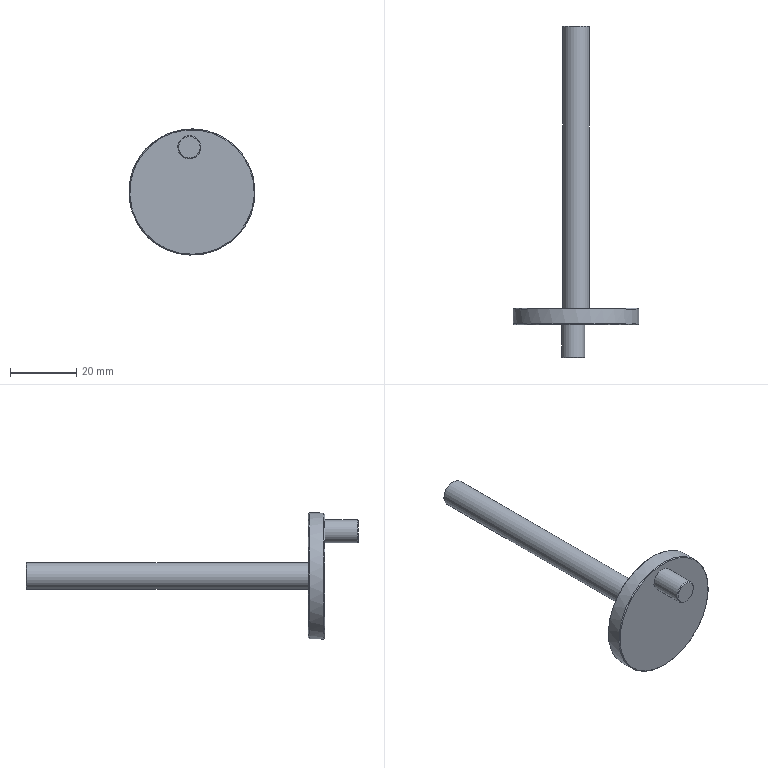Component | NX | CRANKSHAFT | 1 solid | 11 faces | box 38 x 100 x 38 mm | volume 10319 mm3 | plane 4 | cone 4 | cylinder 3 | commonest cylinder face diameters 38 x1 8 x1 7 x1
STEP:
#1=CARTESIAN_POINT('',(0.,0.,0.));
#2=DIRECTION('',(0.,0.,1.));
#3=DIRECTION('',(1.,0.,0.));
#4=AXIS2_PLACEMENT_3D('',#1,#2,#3);
#5=CARTESIAN_POINT('',(18.717,-24.75,42.11));
#6=VERTEX_POINT('',#5);
#7=CARTESIAN_POINT('',(0.,-24.75,41.));
#8=DIRECTION('',(0.,1.,0.));
#9=DIRECTION('',(0.9982,0.,0.05921));
#10=AXIS2_PLACEMENT_3D('',#7,#8,#9);
#11=CIRCLE('',#10,18.75);
#12=CARTESIAN_POINT('',(0.,-24.75,41.));
#13=DIRECTION('',(0.,1.,0.));
#14=DIRECTION('',(0.9982,0.,0.05921));
#15=AXIS2_PLACEMENT_3D('',#12,#13,#14);
#16=PLANE('',#15);
#17=CARTESIAN_POINT('',(0.,0.));
#18=DIRECTION('',(1.,0.));
#19=AXIS2_PLACEMENT_2D('',#17,#18);
#20=CIRCLE('',#19,18.75);
#21=(GEOMETRIC_REPRESENTATION_CONTEXT(2)PARAMETRIC_REPRESENTATION_CONTEXT()REPRESENTATION_CONTEXT('',''));
#22=DEFINITIONAL_REPRESENTATION('',(#20),#21);
#23=PCURVE('',#16,#22);
#24=CARTESIAN_POINT('',(0.,-25.,41.));
#25=DIRECTION('',(0.,-1.,0.));
#26=DIRECTION('',(-0.9982,0.,-0.05921));
#27=AXIS2_PLACEMENT_3D('',#24,#25,#26);
#28=CONICAL_SURFACE('',#27,19.,0.7854);
#29=CARTESIAN_POINT('',(9.425,-0.25));
#30=DIRECTION('',(-1.,0.));
#31=VECTOR('',#30,1.);
#32=LINE('',#29,#31);
#33=(GEOMETRIC_REPRESENTATION_CONTEXT(2)PARAMETRIC_REPRESENTATION_CONTEXT()REPRESENTATION_CONTEXT('',''));
#34=DEFINITIONAL_REPRESENTATION('',(#32),#33);
#35=PCURVE('',#28,#34);
#36=SURFACE_CURVE('',#11,(#23,#35),.PCURVE_S1.);
#37=EDGE_CURVE('',#6,#6,#36,.T.);
#38=ORIENTED_EDGE('',*,*,#37,.T.);
#39=EDGE_LOOP('',(#38));
#40=FACE_BOUND('',#39,.T.);
#41=CARTESIAN_POINT('',(3.993,-24.75,41.237));
#42=VERTEX_POINT('',#41);
#43=CARTESIAN_POINT('',(0.,-24.75,41.));
#44=DIRECTION('',(0.,1.,0.));
#45=DIRECTION('',(0.9982,0.,0.05921));
#46=AXIS2_PLACEMENT_3D('',#43,#44,#45);
#47=CIRCLE('',#46,4.);
#48=CARTESIAN_POINT('',(-0.,-0.));
#49=DIRECTION('',(1.,-0.));
#50=AXIS2_PLACEMENT_2D('',#48,#49);
#51=CIRCLE('',#50,4.);
#52=(GEOMETRIC_REPRESENTATION_CONTEXT(2)PARAMETRIC_REPRESENTATION_CONTEXT()REPRESENTATION_CONTEXT('',''));
#53=DEFINITIONAL_REPRESENTATION('',(#51),#52);
#54=PCURVE('',#16,#53);
#55=CARTESIAN_POINT('',(0.,-24.75,41.));
#56=DIRECTION('',(0.,1.,0.));
#57=DIRECTION('',(0.9982,0.,0.05921));
#58=AXIS2_PLACEMENT_3D('',#55,#56,#57);
#59=CYLINDRICAL_SURFACE('',#58,4.);
#60=CARTESIAN_POINT('',(0.,0.));
#61=DIRECTION('',(1.,0.));
#62=VECTOR('',#61,1.);
#63=LINE('',#60,#62);
#64=(GEOMETRIC_REPRESENTATION_CONTEXT(2)PARAMETRIC_REPRESENTATION_CONTEXT()REPRESENTATION_CONTEXT('',''));
#65=DEFINITIONAL_REPRESENTATION('',(#63),#64);
#66=PCURVE('',#59,#65);
#67=SURFACE_CURVE('',#47,(#54,#66),.PCURVE_S1.);
#68=EDGE_CURVE('',#42,#42,#67,.T.);
#69=ORIENTED_EDGE('',*,*,#68,.F.);
#70=EDGE_LOOP('',(#69));
#71=FACE_BOUND('',#70,.T.);
#72=ADVANCED_FACE('',(#40,#71),#16,.T.);
#73=CARTESIAN_POINT('',(-18.717,-29.75,39.89));
#74=VERTEX_POINT('',#73);
#75=CARTESIAN_POINT('',(0.,-29.75,41.));
#76=DIRECTION('',(0.,-1.,0.));
#77=DIRECTION('',(-0.9982,0.,-0.05921));
#78=AXIS2_PLACEMENT_3D('',#75,#76,#77);
#79=CIRCLE('',#78,18.75);
#80=CARTESIAN_POINT('',(0.,-29.75,41.));
#81=DIRECTION('',(0.,-1.,0.));
#82=DIRECTION('',(-0.9982,0.,-0.05921));
#83=AXIS2_PLACEMENT_3D('',#80,#81,#82);
#84=PLANE('',#83);
#85=CARTESIAN_POINT('',(0.,0.));
#86=DIRECTION('',(1.,0.));
#87=AXIS2_PLACEMENT_2D('',#85,#86);
#88=CIRCLE('',#87,18.75);
#89=(GEOMETRIC_REPRESENTATION_CONTEXT(2)PARAMETRIC_REPRESENTATION_CONTEXT()REPRESENTATION_CONTEXT('',''));
#90=DEFINITIONAL_REPRESENTATION('',(#88),#89);
#91=PCURVE('',#84,#90);
#92=CARTESIAN_POINT('',(0.,-29.5,41.));
#93=DIRECTION('',(0.,1.,0.));
#94=DIRECTION('',(0.9982,0.,0.05921));
#95=AXIS2_PLACEMENT_3D('',#92,#93,#94);
#96=CONICAL_SURFACE('',#95,19.,0.7854);
#97=CARTESIAN_POINT('',(9.425,-0.25));
#98=DIRECTION('',(-1.,0.));
#99=VECTOR('',#98,1.);
#100=LINE('',#97,#99);
#101=(GEOMETRIC_REPRESENTATION_CONTEXT(2)PARAMETRIC_REPRESENTATION_CONTEXT()REPRESENTATION_CONTEXT('',''));
#102=DEFINITIONAL_REPRESENTATION('',(#100),#101);
#103=PCURVE('',#96,#102);
#104=SURFACE_CURVE('',#79,(#91,#103),.PCURVE_S1.);
#105=EDGE_CURVE('',#74,#74,#104,.T.);
#106=ORIENTED_EDGE('',*,*,#105,.T.);
#107=EDGE_LOOP('',(#106));
#108=FACE_BOUND('',#107,.T.);
#109=CARTESIAN_POINT('',(2.694,-29.75,54.684));
#110=VERTEX_POINT('',#109);
#111=CARTESIAN_POINT('',(-0.7994,-29.75,54.476));
#112=DIRECTION('',(0.,1.,0.));
#113=DIRECTION('',(0.9982,0.,0.05921));
#114=AXIS2_PLACEMENT_3D('',#111,#112,#113);
#115=CIRCLE('',#114,3.5);
#116=CARTESIAN_POINT('',(-3.5,-13.5));
#117=CARTESIAN_POINT('',(-3.5,-7.438));
#118=CARTESIAN_POINT('',(1.75,-10.469));
#119=CARTESIAN_POINT('',(7.,-13.5));
#120=CARTESIAN_POINT('',(1.75,-16.531));
#121=CARTESIAN_POINT('',(-3.5,-19.562));
#122=CARTESIAN_POINT('',(-3.5,-13.5));
#123=(BOUNDED_CURVE()B_SPLINE_CURVE(2,(#116,#117,#118,#119,#120,#121,#122),.UNSPECIFIED.,.T.,.F.)B_SPLINE_CURVE_WITH_KNOTS((1,2,2,2,2,1),(-2.094,0.,2.094,4.189,6.283,8.378),.UNSPECIFIED.)CURVE()GEOMETRIC_REPRESENTATION_ITEM()RATIONAL_B_SPLINE_CURVE((1.,0.5,1.,0.5,1.,0.5,1.))REPRESENTATION_ITEM(''));
#124=(GEOMETRIC_REPRESENTATION_CONTEXT(2)PARAMETRIC_REPRESENTATION_CONTEXT()REPRESENTATION_CONTEXT('',''));
#125=DEFINITIONAL_REPRESENTATION('',(#123),#124);
#126=PCURVE('',#84,#125);
#127=CARTESIAN_POINT('',(-0.7994,-39.75,54.476));
#128=DIRECTION('',(0.,1.,0.));
#129=DIRECTION('',(0.9982,0.,0.05921));
#130=AXIS2_PLACEMENT_3D('',#127,#128,#129);
#131=CYLINDRICAL_SURFACE('',#130,3.5);
#132=CARTESIAN_POINT('',(0.,10.));
#133=DIRECTION('',(1.,0.));
#134=VECTOR('',#133,1.);
#135=LINE('',#132,#134);
#136=(GEOMETRIC_REPRESENTATION_CONTEXT(2)PARAMETRIC_REPRESENTATION_CONTEXT()REPRESENTATION_CONTEXT('',''));
#137=DEFINITIONAL_REPRESENTATION('',(#135),#136);
#138=PCURVE('',#131,#137);
#139=SURFACE_CURVE('',#115,(#126,#138),.PCURVE_S1.);
#140=EDGE_CURVE('',#110,#110,#139,.T.);
#141=ORIENTED_EDGE('',*,*,#140,.T.);
#142=EDGE_LOOP('',(#141));
#143=FACE_BOUND('',#142,.T.);
#144=ADVANCED_FACE('',(#108,#143),#84,.T.);
#145=CARTESIAN_POINT('',(18.967,-25.,42.125));
#146=VERTEX_POINT('',#145);
#147=CARTESIAN_POINT('',(0.,-25.,41.));
#148=DIRECTION('',(0.,-1.,0.));
#149=DIRECTION('',(0.9982,0.,0.05921));
#150=AXIS2_PLACEMENT_3D('',#147,#148,#149);
#151=CIRCLE('',#150,19.);
#152=CARTESIAN_POINT('',(0.,-29.75,41.));
#153=DIRECTION('',(0.,1.,0.));
#154=DIRECTION('',(0.9982,0.,0.05921));
#155=AXIS2_PLACEMENT_3D('',#152,#153,#154);
#156=CYLINDRICAL_SURFACE('',#155,19.);
#157=CARTESIAN_POINT('',(6.283,4.75));
#158=DIRECTION('',(-1.,0.));
#159=VECTOR('',#158,1.);
#160=LINE('',#157,#159);
#161=(GEOMETRIC_REPRESENTATION_CONTEXT(2)PARAMETRIC_REPRESENTATION_CONTEXT()REPRESENTATION_CONTEXT('',''));
#162=DEFINITIONAL_REPRESENTATION('',(#160),#161);
#163=PCURVE('',#156,#162);
#164=CARTESIAN_POINT('',(3.142,0.));
#165=DIRECTION('',(1.,0.));
#166=VECTOR('',#165,1.);
#167=LINE('',#164,#166);
#168=(GEOMETRIC_REPRESENTATION_CONTEXT(2)PARAMETRIC_REPRESENTATION_CONTEXT()REPRESENTATION_CONTEXT('',''));
#169=DEFINITIONAL_REPRESENTATION('',(#167),#168);
#170=PCURVE('',#28,#169);
#171=SURFACE_CURVE('',#151,(#163,#170),.PCURVE_S1.);
#172=EDGE_CURVE('',#146,#146,#171,.T.);
#173=ORIENTED_EDGE('',*,*,#172,.T.);
#174=CARTESIAN_POINT('',(18.967,-29.5,42.125));
#175=VERTEX_POINT('',#174);
#176=CARTESIAN_POINT('',(18.967,-29.5,42.125));
#177=CARTESIAN_POINT('',(18.967,-25.,42.125));
#178=B_SPLINE_CURVE_WITH_KNOTS('',1,(#176,#177),.UNSPECIFIED.,.F.,.F.,(2,2),(0.25,4.75),.PIECEWISE_BEZIER_KNOTS.);
#179=CARTESIAN_POINT('',(0.,0.));
#180=DIRECTION('',(0.,1.));
#181=VECTOR('',#180,1.);
#182=LINE('',#179,#181);
#183=(GEOMETRIC_REPRESENTATION_CONTEXT(2)PARAMETRIC_REPRESENTATION_CONTEXT()REPRESENTATION_CONTEXT('',''));
#184=DEFINITIONAL_REPRESENTATION('',(#182),#183);
#185=PCURVE('',#156,#184);
#186=CARTESIAN_POINT('',(6.283,0.));
#187=DIRECTION('',(0.,1.));
#188=VECTOR('',#187,1.);
#189=LINE('',#186,#188);
#190=(GEOMETRIC_REPRESENTATION_CONTEXT(2)PARAMETRIC_REPRESENTATION_CONTEXT()REPRESENTATION_CONTEXT('',''));
#191=DEFINITIONAL_REPRESENTATION('',(#189),#190);
#192=PCURVE('',#156,#191);
#193=SEAM_CURVE('',#178,(#185,#192),.PCURVE_S1.);
#194=EDGE_CURVE('',#175,#146,#193,.T.);
#195=ORIENTED_EDGE('',*,*,#194,.F.);
#196=CARTESIAN_POINT('',(-18.967,-29.5,39.875));
#197=VERTEX_POINT('',#196);
#198=CARTESIAN_POINT('',(0.,-29.5,41.));
#199=DIRECTION('',(0.,1.,0.));
#200=DIRECTION('',(-0.9982,0.,-0.05921));
#201=AXIS2_PLACEMENT_3D('',#198,#199,#200);
#202=CIRCLE('',#201,19.);
#203=CARTESIAN_POINT('',(-3.142,0.25));
#204=DIRECTION('',(1.,0.));
#205=VECTOR('',#204,1.);
#206=LINE('',#203,#205);
#207=(GEOMETRIC_REPRESENTATION_CONTEXT(2)PARAMETRIC_REPRESENTATION_CONTEXT()REPRESENTATION_CONTEXT('',''));
#208=DEFINITIONAL_REPRESENTATION('',(#206),#207);
#209=PCURVE('',#156,#208);
#210=CARTESIAN_POINT('',(3.142,0.));
#211=DIRECTION('',(1.,0.));
#212=VECTOR('',#211,1.);
#213=LINE('',#210,#212);
#214=(GEOMETRIC_REPRESENTATION_CONTEXT(2)PARAMETRIC_REPRESENTATION_CONTEXT()REPRESENTATION_CONTEXT('',''));
#215=DEFINITIONAL_REPRESENTATION('',(#213),#214);
#216=PCURVE('',#96,#215);
#217=SURFACE_CURVE('',#202,(#209,#216),.PCURVE_S1.);
#218=EDGE_CURVE('',#175,#197,#217,.T.);
#219=ORIENTED_EDGE('',*,*,#218,.T.);
#220=CARTESIAN_POINT('',(0.,-29.5,41.));
#221=DIRECTION('',(0.,1.,0.));
#222=DIRECTION('',(-0.9982,0.,-0.05921));
#223=AXIS2_PLACEMENT_3D('',#220,#221,#222);
#224=CIRCLE('',#223,19.);
#225=CARTESIAN_POINT('',(3.142,0.25));
#226=DIRECTION('',(1.,0.));
#227=VECTOR('',#226,1.);
#228=LINE('',#225,#227);
#229=(GEOMETRIC_REPRESENTATION_CONTEXT(2)PARAMETRIC_REPRESENTATION_CONTEXT()REPRESENTATION_CONTEXT('',''));
#230=DEFINITIONAL_REPRESENTATION('',(#228),#229);
#231=PCURVE('',#156,#230);
#232=CARTESIAN_POINT('',(3.142,0.));
#233=DIRECTION('',(1.,-0.));
#234=VECTOR('',#233,1.);
#235=LINE('',#232,#234);
#236=(GEOMETRIC_REPRESENTATION_CONTEXT(2)PARAMETRIC_REPRESENTATION_CONTEXT()REPRESENTATION_CONTEXT('',''));
#237=DEFINITIONAL_REPRESENTATION('',(#235),#236);
#238=PCURVE('',#96,#237);
#239=SURFACE_CURVE('',#224,(#231,#238),.PCURVE_S1.);
#240=EDGE_CURVE('',#197,#175,#239,.T.);
#241=ORIENTED_EDGE('',*,*,#240,.T.);
#242=ORIENTED_EDGE('',*,*,#194,.T.);
#243=EDGE_LOOP('',(#173,#195,#219,#241,#242));
#244=FACE_BOUND('',#243,.T.);
#245=ADVANCED_FACE('',(#244),#156,.T.);
#246=CARTESIAN_POINT('',(3.743,60.25,41.222));
#247=VERTEX_POINT('',#246);
#248=CARTESIAN_POINT('',(0.,60.25,41.));
#249=DIRECTION('',(0.,1.,0.));
#250=DIRECTION('',(0.9982,0.,0.05921));
#251=AXIS2_PLACEMENT_3D('',#248,#249,#250);
#252=CIRCLE('',#251,3.75);
#253=CARTESIAN_POINT('',(0.,60.25,41.));
#254=DIRECTION('',(0.,1.,0.));
#255=DIRECTION('',(0.9982,0.,0.05921));
#256=AXIS2_PLACEMENT_3D('',#253,#254,#255);
#257=PLANE('',#256);
#258=CARTESIAN_POINT('',(0.,0.));
#259=DIRECTION('',(1.,-0.));
#260=AXIS2_PLACEMENT_2D('',#258,#259);
#261=CIRCLE('',#260,3.75);
#262=(GEOMETRIC_REPRESENTATION_CONTEXT(2)PARAMETRIC_REPRESENTATION_CONTEXT()REPRESENTATION_CONTEXT('',''));
#263=DEFINITIONAL_REPRESENTATION('',(#261),#262);
#264=PCURVE('',#257,#263);
#265=CARTESIAN_POINT('',(0.,60.25,41.));
#266=DIRECTION('',(0.,-1.,0.));
#267=DIRECTION('',(-0.9982,0.,-0.05921));
#268=AXIS2_PLACEMENT_3D('',#265,#266,#267);
#269=CONICAL_SURFACE('',#268,3.75,0.7854);
#270=CARTESIAN_POINT('',(9.425,0.));
#271=DIRECTION('',(-1.,0.));
#272=VECTOR('',#271,1.);
#273=LINE('',#270,#272);
#274=(GEOMETRIC_REPRESENTATION_CONTEXT(2)PARAMETRIC_REPRESENTATION_CONTEXT()REPRESENTATION_CONTEXT('',''));
#275=DEFINITIONAL_REPRESENTATION('',(#273),#274);
#276=PCURVE('',#269,#275);
#277=SURFACE_CURVE('',#252,(#264,#276),.PCURVE_S1.);
#278=EDGE_CURVE('',#247,#247,#277,.T.);
#279=ORIENTED_EDGE('',*,*,#278,.T.);
#280=EDGE_LOOP('',(#279));
#281=FACE_BOUND('',#280,.T.);
#282=ADVANCED_FACE('',(#281),#257,.T.);
#283=CARTESIAN_POINT('',(3.993,60.,41.237));
#284=VERTEX_POINT('',#283);
#285=CARTESIAN_POINT('',(0.,60.,41.));
#286=DIRECTION('',(0.,-1.,0.));
#287=DIRECTION('',(0.9982,0.,0.05921));
#288=AXIS2_PLACEMENT_3D('',#285,#286,#287);
#289=CIRCLE('',#288,4.);
#290=CARTESIAN_POINT('',(6.283,84.75));
#291=DIRECTION('',(-1.,0.));
#292=VECTOR('',#291,1.);
#293=LINE('',#290,#292);
#294=(GEOMETRIC_REPRESENTATION_CONTEXT(2)PARAMETRIC_REPRESENTATION_CONTEXT()REPRESENTATION_CONTEXT('',''));
#295=DEFINITIONAL_REPRESENTATION('',(#293),#294);
#296=PCURVE('',#59,#295);
#297=CARTESIAN_POINT('',(3.142,0.25));
#298=DIRECTION('',(1.,0.));
#299=VECTOR('',#298,1.);
#300=LINE('',#297,#299);
#301=(GEOMETRIC_REPRESENTATION_CONTEXT(2)PARAMETRIC_REPRESENTATION_CONTEXT()REPRESENTATION_CONTEXT('',''));
#302=DEFINITIONAL_REPRESENTATION('',(#300),#301);
#303=PCURVE('',#269,#302);
#304=SURFACE_CURVE('',#289,(#296,#303),.PCURVE_S1.);
#305=EDGE_CURVE('',#284,#284,#304,.T.);
#306=ORIENTED_EDGE('',*,*,#305,.T.);
#307=CARTESIAN_POINT('',(3.993,-24.75,41.237));
#308=CARTESIAN_POINT('',(3.993,60.,41.237));
#309=B_SPLINE_CURVE_WITH_KNOTS('',1,(#307,#308),.UNSPECIFIED.,.F.,.F.,(2,2),(0.,84.75),.PIECEWISE_BEZIER_KNOTS.);
#310=CARTESIAN_POINT('',(0.,0.));
#311=DIRECTION('',(0.,1.));
#312=VECTOR('',#311,1.);
#313=LINE('',#310,#312);
#314=(GEOMETRIC_REPRESENTATION_CONTEXT(2)PARAMETRIC_REPRESENTATION_CONTEXT()REPRESENTATION_CONTEXT('',''));
#315=DEFINITIONAL_REPRESENTATION('',(#313),#314);
#316=PCURVE('',#59,#315);
#317=CARTESIAN_POINT('',(6.283,0.));
#318=DIRECTION('',(0.,1.));
#319=VECTOR('',#318,1.);
#320=LINE('',#317,#319);
#321=(GEOMETRIC_REPRESENTATION_CONTEXT(2)PARAMETRIC_REPRESENTATION_CONTEXT()REPRESENTATION_CONTEXT('',''));
#322=DEFINITIONAL_REPRESENTATION('',(#320),#321);
#323=PCURVE('',#59,#322);
#324=SEAM_CURVE('',#309,(#316,#323),.PCURVE_S1.);
#325=EDGE_CURVE('',#42,#284,#324,.T.);
#326=ORIENTED_EDGE('',*,*,#325,.F.);
#327=ORIENTED_EDGE('',*,*,#68,.T.);
#328=ORIENTED_EDGE('',*,*,#325,.T.);
#329=EDGE_LOOP('',(#306,#326,#327,#328));
#330=FACE_BOUND('',#329,.T.);
#331=ADVANCED_FACE('',(#330),#59,.T.);
#332=CARTESIAN_POINT('',(2.694,-39.5,54.684));
#333=VERTEX_POINT('',#332);
#334=CARTESIAN_POINT('',(-0.7994,-39.5,54.476));
#335=DIRECTION('',(0.,1.,0.));
#336=DIRECTION('',(0.9982,0.,0.05921));
#337=AXIS2_PLACEMENT_3D('',#334,#335,#336);
#338=CIRCLE('',#337,3.5);
#339=CARTESIAN_POINT('',(0.,0.25));
#340=DIRECTION('',(1.,0.));
#341=VECTOR('',#340,1.);
#342=LINE('',#339,#341);
#343=(GEOMETRIC_REPRESENTATION_CONTEXT(2)PARAMETRIC_REPRESENTATION_CONTEXT()REPRESENTATION_CONTEXT('',''));
#344=DEFINITIONAL_REPRESENTATION('',(#342),#343);
#345=PCURVE('',#131,#344);
#346=CARTESIAN_POINT('',(-0.7994,-39.5,54.476));
#347=DIRECTION('',(0.,1.,0.));
#348=DIRECTION('',(0.9982,0.,0.05921));
#349=AXIS2_PLACEMENT_3D('',#346,#347,#348);
#350=CONICAL_SURFACE('',#349,3.5,0.7854);
#351=CARTESIAN_POINT('',(0.,0.));
#352=DIRECTION('',(1.,0.));
#353=VECTOR('',#352,1.);
#354=LINE('',#351,#353);
#355=(GEOMETRIC_REPRESENTATION_CONTEXT(2)PARAMETRIC_REPRESENTATION_CONTEXT()REPRESENTATION_CONTEXT('',''));
#356=DEFINITIONAL_REPRESENTATION('',(#354),#355);
#357=PCURVE('',#350,#356);
#358=SURFACE_CURVE('',#338,(#345,#357),.PCURVE_S1.);
#359=EDGE_CURVE('',#333,#333,#358,.T.);
#360=ORIENTED_EDGE('',*,*,#359,.T.);
#361=CARTESIAN_POINT('',(2.694,-39.5,54.684));
#362=CARTESIAN_POINT('',(2.694,-29.75,54.684));
#363=B_SPLINE_CURVE_WITH_KNOTS('',1,(#361,#362),.UNSPECIFIED.,.F.,.F.,(2,2),(0.25,10.),.PIECEWISE_BEZIER_KNOTS.);
#364=CARTESIAN_POINT('',(6.283,0.));
#365=DIRECTION('',(0.,1.));
#366=VECTOR('',#365,1.);
#367=LINE('',#364,#366);
#368=(GEOMETRIC_REPRESENTATION_CONTEXT(2)PARAMETRIC_REPRESENTATION_CONTEXT()REPRESENTATION_CONTEXT('',''));
#369=DEFINITIONAL_REPRESENTATION('',(#367),#368);
#370=PCURVE('',#131,#369);
#371=CARTESIAN_POINT('',(0.,0.));
#372=DIRECTION('',(0.,1.));
#373=VECTOR('',#372,1.);
#374=LINE('',#371,#373);
#375=(GEOMETRIC_REPRESENTATION_CONTEXT(2)PARAMETRIC_REPRESENTATION_CONTEXT()REPRESENTATION_CONTEXT('',''));
#376=DEFINITIONAL_REPRESENTATION('',(#374),#375);
#377=PCURVE('',#131,#376);
#378=SEAM_CURVE('',#363,(#370,#377),.PCURVE_S1.);
#379=EDGE_CURVE('',#333,#110,#378,.T.);
#380=ORIENTED_EDGE('',*,*,#379,.T.);
#381=ORIENTED_EDGE('',*,*,#140,.F.);
#382=ORIENTED_EDGE('',*,*,#379,.F.);
#383=EDGE_LOOP('',(#360,#380,#381,#382));
#384=FACE_BOUND('',#383,.T.);
#385=ADVANCED_FACE('',(#384),#131,.T.);
#386=CARTESIAN_POINT('',(2.445,-39.75,54.669));
#387=VERTEX_POINT('',#386);
#388=CARTESIAN_POINT('',(-0.7994,-39.75,54.476));
#389=DIRECTION('',(0.,-1.,0.));
#390=DIRECTION('',(0.9982,0.,0.05921));
#391=AXIS2_PLACEMENT_3D('',#388,#389,#390);
#392=CIRCLE('',#391,3.25);
#393=CARTESIAN_POINT('',(-0.7994,-39.75,54.476));
#394=DIRECTION('',(0.,1.,0.));
#395=DIRECTION('',(0.9982,0.,0.05921));
#396=AXIS2_PLACEMENT_3D('',#393,#394,#395);
#397=PLANE('',#396);
#398=CARTESIAN_POINT('',(3.25,-0.));
#399=CARTESIAN_POINT('',(3.25,-5.629));
#400=CARTESIAN_POINT('',(-1.625,-2.815));
#401=CARTESIAN_POINT('',(-6.5,0.));
#402=CARTESIAN_POINT('',(-1.625,2.815));
#403=CARTESIAN_POINT('',(3.25,5.629));
#404=CARTESIAN_POINT('',(3.25,-0.));
#405=(BOUNDED_CURVE()B_SPLINE_CURVE(2,(#398,#399,#400,#401,#402,#403,#404),.UNSPECIFIED.,.T.,.F.)B_SPLINE_CURVE_WITH_KNOTS((1,2,2,2,2,1),(-2.094,0.,2.094,4.189,6.283,8.378),.UNSPECIFIED.)CURVE()GEOMETRIC_REPRESENTATION_ITEM()RATIONAL_B_SPLINE_CURVE((1.,0.5,1.,0.5,1.,0.5,1.))REPRESENTATION_ITEM(''));
#406=(GEOMETRIC_REPRESENTATION_CONTEXT(2)PARAMETRIC_REPRESENTATION_CONTEXT()REPRESENTATION_CONTEXT('',''));
#407=DEFINITIONAL_REPRESENTATION('',(#405),#406);
#408=PCURVE('',#397,#407);
#409=CARTESIAN_POINT('',(6.283,-0.25));
#410=DIRECTION('',(-1.,0.));
#411=VECTOR('',#410,1.);
#412=LINE('',#409,#411);
#413=(GEOMETRIC_REPRESENTATION_CONTEXT(2)PARAMETRIC_REPRESENTATION_CONTEXT()REPRESENTATION_CONTEXT('',''));
#414=DEFINITIONAL_REPRESENTATION('',(#412),#413);
#415=PCURVE('',#350,#414);
#416=SURFACE_CURVE('',#392,(#408,#415),.PCURVE_S1.);
#417=EDGE_CURVE('',#387,#387,#416,.T.);
#418=ORIENTED_EDGE('',*,*,#417,.T.);
#419=EDGE_LOOP('',(#418));
#420=FACE_BOUND('',#419,.T.);
#421=ADVANCED_FACE('',(#420),#397,.F.);
#422=ORIENTED_EDGE('',*,*,#37,.F.);
#423=CARTESIAN_POINT('',(18.717,-24.75,42.11));
#424=CARTESIAN_POINT('',(18.967,-25.,42.125));
#425=B_SPLINE_CURVE_WITH_KNOTS('',1,(#423,#424),.UNSPECIFIED.,.F.,.F.,(2,2),(-0.3536,0.),.PIECEWISE_BEZIER_KNOTS.);
#426=CARTESIAN_POINT('',(9.425,0.));
#427=DIRECTION('',(0.,1.));
#428=VECTOR('',#427,1.);
#429=LINE('',#426,#428);
#430=(GEOMETRIC_REPRESENTATION_CONTEXT(2)PARAMETRIC_REPRESENTATION_CONTEXT()REPRESENTATION_CONTEXT('',''));
#431=DEFINITIONAL_REPRESENTATION('',(#429),#430);
#432=PCURVE('',#28,#431);
#433=CARTESIAN_POINT('',(3.142,0.));
#434=DIRECTION('',(0.,1.));
#435=VECTOR('',#434,1.);
#436=LINE('',#433,#435);
#437=(GEOMETRIC_REPRESENTATION_CONTEXT(2)PARAMETRIC_REPRESENTATION_CONTEXT()REPRESENTATION_CONTEXT('',''));
#438=DEFINITIONAL_REPRESENTATION('',(#436),#437);
#439=PCURVE('',#28,#438);
#440=SEAM_CURVE('',#425,(#432,#439),.PCURVE_S1.);
#441=EDGE_CURVE('',#6,#146,#440,.T.);
#442=ORIENTED_EDGE('',*,*,#441,.T.);
#443=ORIENTED_EDGE('',*,*,#172,.F.);
#444=ORIENTED_EDGE('',*,*,#441,.F.);
#445=EDGE_LOOP('',(#422,#442,#443,#444));
#446=FACE_BOUND('',#445,.T.);
#447=ADVANCED_FACE('',(#446),#28,.T.);
#448=ORIENTED_EDGE('',*,*,#105,.F.);
#449=CARTESIAN_POINT('',(-18.717,-29.75,39.89));
#450=CARTESIAN_POINT('',(-18.967,-29.5,39.875));
#451=B_SPLINE_CURVE_WITH_KNOTS('',1,(#449,#450),.UNSPECIFIED.,.F.,.F.,(2,2),(-0.3536,0.),.PIECEWISE_BEZIER_KNOTS.);
#452=CARTESIAN_POINT('',(9.425,0.));
#453=DIRECTION('',(0.,1.));
#454=VECTOR('',#453,1.);
#455=LINE('',#452,#454);
#456=(GEOMETRIC_REPRESENTATION_CONTEXT(2)PARAMETRIC_REPRESENTATION_CONTEXT()REPRESENTATION_CONTEXT('',''));
#457=DEFINITIONAL_REPRESENTATION('',(#455),#456);
#458=PCURVE('',#96,#457);
#459=CARTESIAN_POINT('',(3.142,0.));
#460=DIRECTION('',(0.,1.));
#461=VECTOR('',#460,1.);
#462=LINE('',#459,#461);
#463=(GEOMETRIC_REPRESENTATION_CONTEXT(2)PARAMETRIC_REPRESENTATION_CONTEXT()REPRESENTATION_CONTEXT('',''));
#464=DEFINITIONAL_REPRESENTATION('',(#462),#463);
#465=PCURVE('',#96,#464);
#466=SEAM_CURVE('',#451,(#458,#465),.PCURVE_S1.);
#467=EDGE_CURVE('',#74,#197,#466,.T.);
#468=ORIENTED_EDGE('',*,*,#467,.T.);
#469=ORIENTED_EDGE('',*,*,#218,.F.);
#470=ORIENTED_EDGE('',*,*,#240,.F.);
#471=ORIENTED_EDGE('',*,*,#467,.F.);
#472=EDGE_LOOP('',(#448,#468,#469,#470,#471));
#473=FACE_BOUND('',#472,.T.);
#474=ADVANCED_FACE('',(#473),#96,.T.);
#475=ORIENTED_EDGE('',*,*,#305,.F.);
#476=CARTESIAN_POINT('',(3.743,60.25,41.222));
#477=CARTESIAN_POINT('',(3.993,60.,41.237));
#478=B_SPLINE_CURVE_WITH_KNOTS('',1,(#476,#477),.UNSPECIFIED.,.F.,.F.,(2,2),(0.,0.3536),.PIECEWISE_BEZIER_KNOTS.);
#479=CARTESIAN_POINT('',(3.142,0.));
#480=DIRECTION('',(0.,1.));
#481=VECTOR('',#480,1.);
#482=LINE('',#479,#481);
#483=(GEOMETRIC_REPRESENTATION_CONTEXT(2)PARAMETRIC_REPRESENTATION_CONTEXT()REPRESENTATION_CONTEXT('',''));
#484=DEFINITIONAL_REPRESENTATION('',(#482),#483);
#485=PCURVE('',#269,#484);
#486=CARTESIAN_POINT('',(9.425,0.));
#487=DIRECTION('',(0.,1.));
#488=VECTOR('',#487,1.);
#489=LINE('',#486,#488);
#490=(GEOMETRIC_REPRESENTATION_CONTEXT(2)PARAMETRIC_REPRESENTATION_CONTEXT()REPRESENTATION_CONTEXT('',''));
#491=DEFINITIONAL_REPRESENTATION('',(#489),#490);
#492=PCURVE('',#269,#491);
#493=SEAM_CURVE('',#478,(#485,#492),.PCURVE_S1.);
#494=EDGE_CURVE('',#247,#284,#493,.T.);
#495=ORIENTED_EDGE('',*,*,#494,.F.);
#496=ORIENTED_EDGE('',*,*,#278,.F.);
#497=ORIENTED_EDGE('',*,*,#494,.T.);
#498=EDGE_LOOP('',(#475,#495,#496,#497));
#499=FACE_BOUND('',#498,.T.);
#500=ADVANCED_FACE('',(#499),#269,.T.);
#501=ORIENTED_EDGE('',*,*,#417,.F.);
#502=CARTESIAN_POINT('',(2.445,-39.75,54.669));
#503=CARTESIAN_POINT('',(2.694,-39.5,54.684));
#504=B_SPLINE_CURVE_WITH_KNOTS('',1,(#502,#503),.UNSPECIFIED.,.F.,.F.,(2,2),(-0.3536,0.),.PIECEWISE_BEZIER_KNOTS.);
#505=CARTESIAN_POINT('',(6.283,0.));
#506=DIRECTION('',(0.,1.));
#507=VECTOR('',#506,1.);
#508=LINE('',#505,#507);
#509=(GEOMETRIC_REPRESENTATION_CONTEXT(2)PARAMETRIC_REPRESENTATION_CONTEXT()REPRESENTATION_CONTEXT('',''));
#510=DEFINITIONAL_REPRESENTATION('',(#508),#509);
#511=PCURVE('',#350,#510);
#512=CARTESIAN_POINT('',(0.,0.));
#513=DIRECTION('',(0.,1.));
#514=VECTOR('',#513,1.);
#515=LINE('',#512,#514);
#516=(GEOMETRIC_REPRESENTATION_CONTEXT(2)PARAMETRIC_REPRESENTATION_CONTEXT()REPRESENTATION_CONTEXT('',''));
#517=DEFINITIONAL_REPRESENTATION('',(#515),#516);
#518=PCURVE('',#350,#517);
#519=SEAM_CURVE('',#504,(#511,#518),.PCURVE_S1.);
#520=EDGE_CURVE('',#387,#333,#519,.T.);
#521=ORIENTED_EDGE('',*,*,#520,.T.);
#522=ORIENTED_EDGE('',*,*,#359,.F.);
#523=ORIENTED_EDGE('',*,*,#520,.F.);
#524=EDGE_LOOP('',(#501,#521,#522,#523));
#525=FACE_BOUND('',#524,.T.);
#526=ADVANCED_FACE('',(#525),#350,.T.);
#527=CLOSED_SHELL('',(#72,#144,#245,#282,#331,#385,#421,#447,#474,#500,#526));
#528=MANIFOLD_SOLID_BREP('',#527);
#529=(LENGTH_UNIT()NAMED_UNIT(*)SI_UNIT(.MILLI.,.METRE.));
#530=UNCERTAINTY_MEASURE_WITH_UNIT(LENGTH_MEASURE(0.00001),#529,'','');
#531=(NAMED_UNIT(*)PLANE_ANGLE_UNIT()SI_UNIT($,.RADIAN.));
#532=(NAMED_UNIT(*)SI_UNIT($,.STERADIAN.)SOLID_ANGLE_UNIT());
#533=(GEOMETRIC_REPRESENTATION_CONTEXT(3)GLOBAL_UNCERTAINTY_ASSIGNED_CONTEXT((#530))GLOBAL_UNIT_ASSIGNED_CONTEXT((#529,#531,#532))REPRESENTATION_CONTEXT('',''));
#534=ADVANCED_BREP_SHAPE_REPRESENTATION('',(#4,#528),#533);